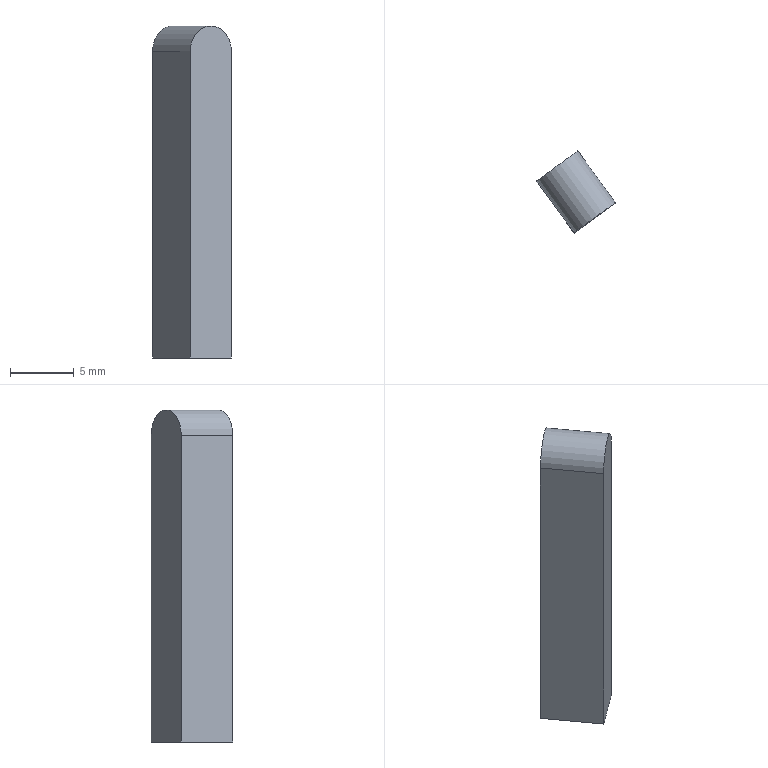Component | SolidWorks | XT-1-16-2-1 | 1 solid | 6 faces | box 6.18 x 6.4 x 26 mm | volume 511 mm3 | plane 5 | cylinder 1 | commonest cylinder face diameters 4 x1
build123d program:
from build123d import *

# Parameters (mm, degrees)
BOSS_EXTRUDE1_DEPTH = 5


with BuildPart() as part:
    # Sketch1 → Boss-Extrude1 (new body)
    with BuildSketch(Plane.XY):
        with BuildLine():
            Line((0, 0), (0, -24))
            Line((0, -24), (4, -24))
            Line((4, -24), (4, 0))
            ThreePointArc((4, 0), (2, 2), (0, 0))
        make_face()
    extrude(amount=BOSS_EXTRUDE1_DEPTH)


solid = part.part

# Placed as in the assembly
solid = solid.moved(Location((498.748, -229.801, -175), (-90, -36.094, -180)))
STEP:
#1=COLOUR_RGB('',0.7922,0.8196,0.9333);
#2=FILL_AREA_STYLE_COLOUR('',#1);
#3=FILL_AREA_STYLE('',(#2));
#4=SURFACE_STYLE_FILL_AREA(#3);
#5=SURFACE_SIDE_STYLE('',(#4));
#6=SURFACE_STYLE_USAGE(.BOTH.,#5);
#7=PRESENTATION_STYLE_ASSIGNMENT((#6));
#8=CARTESIAN_POINT('',(19.509,-9.14,-6.89));
#9=VERTEX_POINT('',#8);
#10=CARTESIAN_POINT('',(19.636,-9.047,-6.89));
#11=VERTEX_POINT('',#10);
#12=CARTESIAN_POINT('',(19.572,-9.094,-6.89));
#13=DIRECTION('',(-0.5891,0.8081,-0.));
#14=DIRECTION('',(0.8081,0.5891,0.));
#15=AXIS2_PLACEMENT_3D('',#12,#13,#14);
#16=CIRCLE('',#15,0.07874);
#17=EDGE_CURVE('',#9,#11,#16,.T.);
#18=ORIENTED_EDGE('',*,*,#17,.T.);
#19=CARTESIAN_POINT('',(19.52,-8.888,-6.89));
#20=VERTEX_POINT('',#19);
#21=CARTESIAN_POINT('',(19.52,-8.888,-6.89));
#22=DIRECTION('',(0.5891,-0.8081,0.));
#23=VECTOR('',#22,39.37);
#24=LINE('',#21,#23);
#25=EDGE_CURVE('',#20,#11,#24,.T.);
#26=ORIENTED_EDGE('',*,*,#25,.F.);
#27=CARTESIAN_POINT('',(19.393,-8.981,-6.89));
#28=VERTEX_POINT('',#27);
#29=CARTESIAN_POINT('',(19.456,-8.935,-6.89));
#30=DIRECTION('',(-0.5891,0.8081,-0.));
#31=DIRECTION('',(0.8081,0.5891,0.));
#32=AXIS2_PLACEMENT_3D('',#29,#30,#31);
#33=CIRCLE('',#32,0.07874);
#34=EDGE_CURVE('',#28,#20,#33,.T.);
#35=ORIENTED_EDGE('',*,*,#34,.F.);
#36=CARTESIAN_POINT('',(19.393,-8.981,-6.89));
#37=DIRECTION('',(0.5891,-0.8081,0.));
#38=VECTOR('',#37,39.37);
#39=LINE('',#36,#38);
#40=EDGE_CURVE('',#28,#9,#39,.T.);
#41=ORIENTED_EDGE('',*,*,#40,.T.);
#42=EDGE_LOOP('',(#18,#26,#35,#41));
#43=FACE_OUTER_BOUND('',#42,.T.);
#44=CARTESIAN_POINT('',(19.456,-8.935,-6.89));
#45=DIRECTION('',(0.5891,-0.8081,0.));
#46=DIRECTION('',(0.8081,0.5891,0.));
#47=AXIS2_PLACEMENT_3D('',#44,#45,#46);
#48=CYLINDRICAL_SURFACE('',#47,0.07874);
#49=ADVANCED_FACE('',(#43),#48,.T.);
#50=CARTESIAN_POINT('',(19.636,-9.047,-7.835));
#51=VERTEX_POINT('',#50);
#52=CARTESIAN_POINT('',(19.636,-9.047,-6.89));
#53=DIRECTION('',(0.,-0.,-1.));
#54=VECTOR('',#53,39.37);
#55=LINE('',#52,#54);
#56=EDGE_CURVE('',#11,#51,#55,.T.);
#57=ORIENTED_EDGE('',*,*,#56,.T.);
#58=CARTESIAN_POINT('',(19.52,-8.888,-7.835));
#59=VERTEX_POINT('',#58);
#60=CARTESIAN_POINT('',(19.52,-8.888,-7.835));
#61=DIRECTION('',(0.5891,-0.8081,0.));
#62=VECTOR('',#61,39.37);
#63=LINE('',#60,#62);
#64=EDGE_CURVE('',#59,#51,#63,.T.);
#65=ORIENTED_EDGE('',*,*,#64,.F.);
#66=CARTESIAN_POINT('',(19.52,-8.888,-6.89));
#67=DIRECTION('',(0.,-0.,-1.));
#68=VECTOR('',#67,39.37);
#69=LINE('',#66,#68);
#70=EDGE_CURVE('',#20,#59,#69,.T.);
#71=ORIENTED_EDGE('',*,*,#70,.F.);
#72=ORIENTED_EDGE('',*,*,#25,.T.);
#73=EDGE_LOOP('',(#57,#65,#71,#72));
#74=FACE_OUTER_BOUND('',#73,.T.);
#75=CARTESIAN_POINT('',(19.52,-8.888,-6.89));
#76=DIRECTION('',(-0.8081,-0.5891,-0.));
#77=DIRECTION('',(-0.,0.,1.));
#78=AXIS2_PLACEMENT_3D('',#75,#76,#77);
#79=PLANE('',#78);
#80=ADVANCED_FACE('',(#74),#79,.F.);
#81=CARTESIAN_POINT('',(19.509,-9.14,-7.835));
#82=VERTEX_POINT('',#81);
#83=CARTESIAN_POINT('',(19.636,-9.047,-7.835));
#84=DIRECTION('',(-0.8081,-0.5891,-0.));
#85=VECTOR('',#84,39.37);
#86=LINE('',#83,#85);
#87=EDGE_CURVE('',#51,#82,#86,.T.);
#88=ORIENTED_EDGE('',*,*,#87,.T.);
#89=CARTESIAN_POINT('',(19.393,-8.981,-7.835));
#90=VERTEX_POINT('',#89);
#91=CARTESIAN_POINT('',(19.393,-8.981,-7.835));
#92=DIRECTION('',(0.5891,-0.8081,0.));
#93=VECTOR('',#92,39.37);
#94=LINE('',#91,#93);
#95=EDGE_CURVE('',#90,#82,#94,.T.);
#96=ORIENTED_EDGE('',*,*,#95,.F.);
#97=CARTESIAN_POINT('',(19.52,-8.888,-7.835));
#98=DIRECTION('',(-0.8081,-0.5891,-0.));
#99=VECTOR('',#98,39.37);
#100=LINE('',#97,#99);
#101=EDGE_CURVE('',#59,#90,#100,.T.);
#102=ORIENTED_EDGE('',*,*,#101,.F.);
#103=ORIENTED_EDGE('',*,*,#64,.T.);
#104=EDGE_LOOP('',(#88,#96,#102,#103));
#105=FACE_OUTER_BOUND('',#104,.T.);
#106=CARTESIAN_POINT('',(19.52,-8.888,-7.835));
#107=DIRECTION('',(-0.,0.,1.));
#108=DIRECTION('',(-0.5891,0.8081,-0.));
#109=AXIS2_PLACEMENT_3D('',#106,#107,#108);
#110=PLANE('',#109);
#111=ADVANCED_FACE('',(#105),#110,.F.);
#112=CARTESIAN_POINT('',(19.509,-9.14,-6.89));
#113=DIRECTION('',(-0.,0.,1.));
#114=VECTOR('',#113,39.37);
#115=LINE('',#112,#114);
#116=EDGE_CURVE('',#82,#9,#115,.T.);
#117=ORIENTED_EDGE('',*,*,#116,.T.);
#118=ORIENTED_EDGE('',*,*,#40,.F.);
#119=CARTESIAN_POINT('',(19.393,-8.981,-6.89));
#120=DIRECTION('',(-0.,0.,1.));
#121=VECTOR('',#120,39.37);
#122=LINE('',#119,#121);
#123=EDGE_CURVE('',#90,#28,#122,.T.);
#124=ORIENTED_EDGE('',*,*,#123,.F.);
#125=ORIENTED_EDGE('',*,*,#95,.T.);
#126=EDGE_LOOP('',(#117,#118,#124,#125));
#127=FACE_OUTER_BOUND('',#126,.T.);
#128=CARTESIAN_POINT('',(19.393,-8.981,-6.89));
#129=DIRECTION('',(0.8081,0.5891,0.));
#130=DIRECTION('',(0.,-0.,-1.));
#131=AXIS2_PLACEMENT_3D('',#128,#129,#130);
#132=PLANE('',#131);
#133=ADVANCED_FACE('',(#127),#132,.F.);
#134=ORIENTED_EDGE('',*,*,#34,.T.);
#135=ORIENTED_EDGE('',*,*,#70,.T.);
#136=ORIENTED_EDGE('',*,*,#101,.T.);
#137=ORIENTED_EDGE('',*,*,#123,.T.);
#138=EDGE_LOOP('',(#134,#135,#136,#137));
#139=FACE_OUTER_BOUND('',#138,.T.);
#140=CARTESIAN_POINT('',(19.456,-8.935,-6.89));
#141=DIRECTION('',(0.5891,-0.8081,0.));
#142=DIRECTION('',(0.8081,0.5891,0.));
#143=AXIS2_PLACEMENT_3D('',#140,#141,#142);
#144=PLANE('',#143);
#145=ADVANCED_FACE('',(#139),#144,.F.);
#146=ORIENTED_EDGE('',*,*,#17,.F.);
#147=ORIENTED_EDGE('',*,*,#116,.F.);
#148=ORIENTED_EDGE('',*,*,#87,.F.);
#149=ORIENTED_EDGE('',*,*,#56,.F.);
#150=EDGE_LOOP('',(#146,#147,#148,#149));
#151=FACE_OUTER_BOUND('',#150,.T.);
#152=CARTESIAN_POINT('',(19.572,-9.094,-6.89));
#153=DIRECTION('',(0.5891,-0.8081,0.));
#154=DIRECTION('',(0.8081,0.5891,0.));
#155=AXIS2_PLACEMENT_3D('',#152,#153,#154);
#156=PLANE('',#155);
#157=ADVANCED_FACE('',(#151),#156,.T.);
#158=CLOSED_SHELL('',(#49,#80,#111,#133,#145,#157));
#159=MANIFOLD_SOLID_BREP('',#158);
#160=STYLED_ITEM('',(#7),#159);
#161=PRESENTATION_LAYER_ASSIGNMENT('','',(#160));
#162=(LENGTH_UNIT()NAMED_UNIT(*)SI_UNIT($,.METRE.));
#163=LENGTH_MEASURE_WITH_UNIT(LENGTH_MEASURE(0.0254),#162);
#164=DIMENSIONAL_EXPONENTS(1.,0.,0.,0.,0.,0.,0.);
#165=(CONVERSION_BASED_UNIT('',#163)LENGTH_UNIT()NAMED_UNIT(#164));
#166=UNCERTAINTY_MEASURE_WITH_UNIT(LENGTH_MEASURE(0.00001),#165,'','');
#167=(NAMED_UNIT(*)PLANE_ANGLE_UNIT()SI_UNIT($,.RADIAN.));
#168=(NAMED_UNIT(*)SI_UNIT($,.STERADIAN.)SOLID_ANGLE_UNIT());
#169=(GEOMETRIC_REPRESENTATION_CONTEXT(3)GLOBAL_UNCERTAINTY_ASSIGNED_CONTEXT((#166))GLOBAL_UNIT_ASSIGNED_CONTEXT((#165,#167,#168))REPRESENTATION_CONTEXT('',''));
#170=MECHANICAL_DESIGN_GEOMETRIC_PRESENTATION_REPRESENTATION('',(#160),#169);
#171=CARTESIAN_POINT('',(0.,0.,0.));
#172=DIRECTION('',(0.,0.,1.));
#173=DIRECTION('',(1.,0.,0.));
#174=AXIS2_PLACEMENT_3D('',#171,#172,#173);
#175=(LENGTH_UNIT()NAMED_UNIT(*)SI_UNIT($,.METRE.));
#176=LENGTH_MEASURE_WITH_UNIT(LENGTH_MEASURE(0.0254),#175);
#177=DIMENSIONAL_EXPONENTS(1.,0.,0.,0.,0.,0.,0.);
#178=(CONVERSION_BASED_UNIT('',#176)LENGTH_UNIT()NAMED_UNIT(#177));
#179=UNCERTAINTY_MEASURE_WITH_UNIT(LENGTH_MEASURE(0.00001),#178,'','');
#180=(NAMED_UNIT(*)PLANE_ANGLE_UNIT()SI_UNIT($,.RADIAN.));
#181=(NAMED_UNIT(*)SI_UNIT($,.STERADIAN.)SOLID_ANGLE_UNIT());
#182=(GEOMETRIC_REPRESENTATION_CONTEXT(3)GLOBAL_UNCERTAINTY_ASSIGNED_CONTEXT((#179))GLOBAL_UNIT_ASSIGNED_CONTEXT((#178,#180,#181))REPRESENTATION_CONTEXT('',''));
#183=ADVANCED_BREP_SHAPE_REPRESENTATION('',(#159,#174),#182);